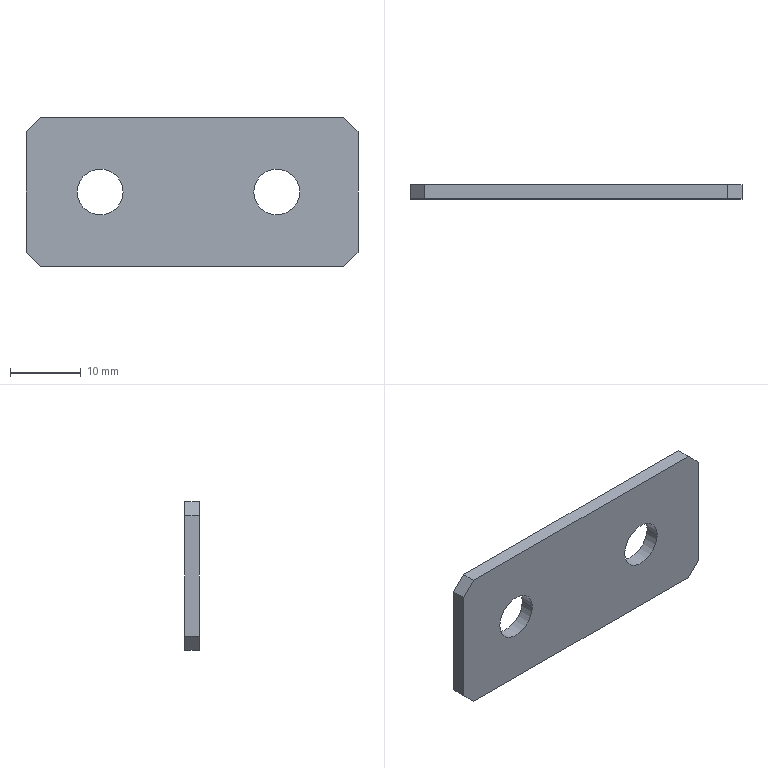Component | SolidWorks | Crossbeam.1(Item52)-1_Block-1 | 1 solid | 14 faces | box 47 x 2 x 21 mm | volume 1825 mm3 | plane 10 | cylinder 4 | commonest cylinder face diameters 6.5 x4 | material Plain Carbon Steel
STEP:
#1=COLOUR_RGB('',0.7922,0.8196,0.9333);
#2=FILL_AREA_STYLE_COLOUR('',#1);
#3=FILL_AREA_STYLE('',(#2));
#4=SURFACE_STYLE_FILL_AREA(#3);
#5=SURFACE_SIDE_STYLE('',(#4));
#6=SURFACE_STYLE_USAGE(.BOTH.,#5);
#7=PRESENTATION_STYLE_ASSIGNMENT((#6));
#8=CARTESIAN_POINT('',(-15.384,14.764,-43.799));
#9=VERTEX_POINT('',#8);
#10=CARTESIAN_POINT('',(-15.128,14.764,-43.799));
#11=VERTEX_POINT('',#10);
#12=CARTESIAN_POINT('',(-15.256,14.764,-43.799));
#13=DIRECTION('',(0.,-1.,-0.));
#14=DIRECTION('',(1.,0.,0.));
#15=AXIS2_PLACEMENT_3D('',#12,#13,#14);
#16=CIRCLE('',#15,0.128);
#17=EDGE_CURVE('',#9,#11,#16,.T.);
#18=ORIENTED_EDGE('',*,*,#17,.F.);
#19=CARTESIAN_POINT('',(-15.384,14.685,-43.799));
#20=VERTEX_POINT('',#19);
#21=CARTESIAN_POINT('',(-15.384,14.764,-43.799));
#22=DIRECTION('',(0.,-1.,-0.));
#23=VECTOR('',#22,39.37);
#24=LINE('',#21,#23);
#25=EDGE_CURVE('',#9,#20,#24,.T.);
#26=ORIENTED_EDGE('',*,*,#25,.T.);
#27=CARTESIAN_POINT('',(-15.128,14.685,-43.799));
#28=VERTEX_POINT('',#27);
#29=CARTESIAN_POINT('',(-15.256,14.685,-43.799));
#30=DIRECTION('',(0.,-1.,-0.));
#31=DIRECTION('',(1.,0.,0.));
#32=AXIS2_PLACEMENT_3D('',#29,#30,#31);
#33=CIRCLE('',#32,0.128);
#34=EDGE_CURVE('',#20,#28,#33,.T.);
#35=ORIENTED_EDGE('',*,*,#34,.T.);
#36=CARTESIAN_POINT('',(-15.128,14.764,-43.799));
#37=DIRECTION('',(0.,-1.,-0.));
#38=VECTOR('',#37,39.37);
#39=LINE('',#36,#38);
#40=EDGE_CURVE('',#11,#28,#39,.T.);
#41=ORIENTED_EDGE('',*,*,#40,.F.);
#42=EDGE_LOOP('',(#18,#26,#35,#41));
#43=FACE_OUTER_BOUND('',#42,.T.);
#44=CARTESIAN_POINT('',(-15.256,14.764,-43.799));
#45=DIRECTION('',(0.,-1.,-0.));
#46=DIRECTION('',(1.,0.,0.));
#47=AXIS2_PLACEMENT_3D('',#44,#45,#46);
#48=CYLINDRICAL_SURFACE('',#47,0.128);
#49=ADVANCED_FACE('',(#43),#48,.F.);
#50=CARTESIAN_POINT('',(-14.4,14.764,-43.799));
#51=VERTEX_POINT('',#50);
#52=CARTESIAN_POINT('',(-14.144,14.764,-43.799));
#53=VERTEX_POINT('',#52);
#54=CARTESIAN_POINT('',(-14.272,14.764,-43.799));
#55=DIRECTION('',(0.,-1.,-0.));
#56=DIRECTION('',(1.,0.,0.));
#57=AXIS2_PLACEMENT_3D('',#54,#55,#56);
#58=CIRCLE('',#57,0.128);
#59=EDGE_CURVE('',#51,#53,#58,.T.);
#60=ORIENTED_EDGE('',*,*,#59,.F.);
#61=CARTESIAN_POINT('',(-14.4,14.685,-43.799));
#62=VERTEX_POINT('',#61);
#63=CARTESIAN_POINT('',(-14.4,14.764,-43.799));
#64=DIRECTION('',(0.,-1.,-0.));
#65=VECTOR('',#64,39.37);
#66=LINE('',#63,#65);
#67=EDGE_CURVE('',#51,#62,#66,.T.);
#68=ORIENTED_EDGE('',*,*,#67,.T.);
#69=CARTESIAN_POINT('',(-14.144,14.685,-43.799));
#70=VERTEX_POINT('',#69);
#71=CARTESIAN_POINT('',(-14.272,14.685,-43.799));
#72=DIRECTION('',(0.,-1.,-0.));
#73=DIRECTION('',(1.,0.,0.));
#74=AXIS2_PLACEMENT_3D('',#71,#72,#73);
#75=CIRCLE('',#74,0.128);
#76=EDGE_CURVE('',#62,#70,#75,.T.);
#77=ORIENTED_EDGE('',*,*,#76,.T.);
#78=CARTESIAN_POINT('',(-14.144,14.764,-43.799));
#79=DIRECTION('',(0.,-1.,-0.));
#80=VECTOR('',#79,39.37);
#81=LINE('',#78,#80);
#82=EDGE_CURVE('',#53,#70,#81,.T.);
#83=ORIENTED_EDGE('',*,*,#82,.F.);
#84=EDGE_LOOP('',(#60,#68,#77,#83));
#85=FACE_OUTER_BOUND('',#84,.T.);
#86=CARTESIAN_POINT('',(-14.272,14.764,-43.799));
#87=DIRECTION('',(0.,-1.,-0.));
#88=DIRECTION('',(1.,0.,0.));
#89=AXIS2_PLACEMENT_3D('',#86,#87,#88);
#90=CYLINDRICAL_SURFACE('',#89,0.128);
#91=ADVANCED_FACE('',(#85),#90,.F.);
#92=CARTESIAN_POINT('',(-13.819,14.764,-44.134));
#93=VERTEX_POINT('',#92);
#94=CARTESIAN_POINT('',(-13.819,14.764,-43.465));
#95=VERTEX_POINT('',#94);
#96=CARTESIAN_POINT('',(-13.819,14.764,-44.213));
#97=DIRECTION('',(-0.,-0.,1.));
#98=VECTOR('',#97,39.37);
#99=LINE('',#96,#98);
#100=EDGE_CURVE('',#93,#95,#99,.T.);
#101=ORIENTED_EDGE('',*,*,#100,.T.);
#102=CARTESIAN_POINT('',(-13.819,14.685,-43.465));
#103=VERTEX_POINT('',#102);
#104=CARTESIAN_POINT('',(-13.819,14.764,-43.465));
#105=DIRECTION('',(0.,-1.,-0.));
#106=VECTOR('',#105,39.37);
#107=LINE('',#104,#106);
#108=EDGE_CURVE('',#95,#103,#107,.T.);
#109=ORIENTED_EDGE('',*,*,#108,.T.);
#110=CARTESIAN_POINT('',(-13.819,14.685,-44.134));
#111=VERTEX_POINT('',#110);
#112=CARTESIAN_POINT('',(-13.819,14.685,-44.213));
#113=DIRECTION('',(-0.,-0.,1.));
#114=VECTOR('',#113,39.37);
#115=LINE('',#112,#114);
#116=EDGE_CURVE('',#111,#103,#115,.T.);
#117=ORIENTED_EDGE('',*,*,#116,.F.);
#118=CARTESIAN_POINT('',(-13.819,14.764,-44.134));
#119=DIRECTION('',(-0.,1.,0.));
#120=VECTOR('',#119,39.37);
#121=LINE('',#118,#120);
#122=EDGE_CURVE('',#111,#93,#121,.T.);
#123=ORIENTED_EDGE('',*,*,#122,.T.);
#124=EDGE_LOOP('',(#101,#109,#117,#123));
#125=FACE_OUTER_BOUND('',#124,.T.);
#126=CARTESIAN_POINT('',(-13.819,14.764,-44.213));
#127=DIRECTION('',(1.,0.,0.));
#128=DIRECTION('',(-0.,1.,0.));
#129=AXIS2_PLACEMENT_3D('',#126,#127,#128);
#130=PLANE('',#129);
#131=ADVANCED_FACE('',(#125),#130,.T.);
#132=CARTESIAN_POINT('',(-15.591,14.685,-44.213));
#133=VERTEX_POINT('',#132);
#134=CARTESIAN_POINT('',(-13.898,14.685,-44.213));
#135=VERTEX_POINT('',#134);
#136=CARTESIAN_POINT('',(-15.669,14.685,-44.213));
#137=DIRECTION('',(1.,0.,0.));
#138=VECTOR('',#137,39.37);
#139=LINE('',#136,#138);
#140=EDGE_CURVE('',#133,#135,#139,.T.);
#141=ORIENTED_EDGE('',*,*,#140,.F.);
#142=CARTESIAN_POINT('',(-15.591,14.764,-44.213));
#143=VERTEX_POINT('',#142);
#144=CARTESIAN_POINT('',(-15.591,14.764,-44.213));
#145=DIRECTION('',(-0.,1.,0.));
#146=VECTOR('',#145,39.37);
#147=LINE('',#144,#146);
#148=EDGE_CURVE('',#133,#143,#147,.T.);
#149=ORIENTED_EDGE('',*,*,#148,.T.);
#150=CARTESIAN_POINT('',(-13.898,14.764,-44.213));
#151=VERTEX_POINT('',#150);
#152=CARTESIAN_POINT('',(-15.669,14.764,-44.213));
#153=DIRECTION('',(1.,0.,0.));
#154=VECTOR('',#153,39.37);
#155=LINE('',#152,#154);
#156=EDGE_CURVE('',#143,#151,#155,.T.);
#157=ORIENTED_EDGE('',*,*,#156,.T.);
#158=CARTESIAN_POINT('',(-13.898,14.764,-44.213));
#159=DIRECTION('',(0.,-1.,-0.));
#160=VECTOR('',#159,39.37);
#161=LINE('',#158,#160);
#162=EDGE_CURVE('',#151,#135,#161,.T.);
#163=ORIENTED_EDGE('',*,*,#162,.T.);
#164=EDGE_LOOP('',(#141,#149,#157,#163));
#165=FACE_OUTER_BOUND('',#164,.T.);
#166=CARTESIAN_POINT('',(-15.669,14.764,-44.213));
#167=DIRECTION('',(0.,0.,-1.));
#168=DIRECTION('',(-0.,1.,0.));
#169=AXIS2_PLACEMENT_3D('',#166,#167,#168);
#170=PLANE('',#169);
#171=ADVANCED_FACE('',(#165),#170,.T.);
#172=CARTESIAN_POINT('',(-15.669,14.685,-43.465));
#173=VERTEX_POINT('',#172);
#174=CARTESIAN_POINT('',(-15.669,14.685,-44.134));
#175=VERTEX_POINT('',#174);
#176=CARTESIAN_POINT('',(-15.669,14.685,-44.213));
#177=DIRECTION('',(0.,0.,-1.));
#178=VECTOR('',#177,39.37);
#179=LINE('',#176,#178);
#180=EDGE_CURVE('',#173,#175,#179,.T.);
#181=ORIENTED_EDGE('',*,*,#180,.F.);
#182=CARTESIAN_POINT('',(-15.669,14.764,-43.465));
#183=VERTEX_POINT('',#182);
#184=CARTESIAN_POINT('',(-15.669,14.764,-43.465));
#185=DIRECTION('',(-0.,1.,0.));
#186=VECTOR('',#185,39.37);
#187=LINE('',#184,#186);
#188=EDGE_CURVE('',#173,#183,#187,.T.);
#189=ORIENTED_EDGE('',*,*,#188,.T.);
#190=CARTESIAN_POINT('',(-15.669,14.764,-44.134));
#191=VERTEX_POINT('',#190);
#192=CARTESIAN_POINT('',(-15.669,14.764,-44.213));
#193=DIRECTION('',(0.,0.,-1.));
#194=VECTOR('',#193,39.37);
#195=LINE('',#192,#194);
#196=EDGE_CURVE('',#183,#191,#195,.T.);
#197=ORIENTED_EDGE('',*,*,#196,.T.);
#198=CARTESIAN_POINT('',(-15.669,14.764,-44.134));
#199=DIRECTION('',(0.,-1.,-0.));
#200=VECTOR('',#199,39.37);
#201=LINE('',#198,#200);
#202=EDGE_CURVE('',#191,#175,#201,.T.);
#203=ORIENTED_EDGE('',*,*,#202,.T.);
#204=EDGE_LOOP('',(#181,#189,#197,#203));
#205=FACE_OUTER_BOUND('',#204,.T.);
#206=CARTESIAN_POINT('',(-15.669,14.764,-44.213));
#207=DIRECTION('',(-1.,-0.,-0.));
#208=DIRECTION('',(0.,-1.,-0.));
#209=AXIS2_PLACEMENT_3D('',#206,#207,#208);
#210=PLANE('',#209);
#211=ADVANCED_FACE('',(#205),#210,.T.);
#212=CARTESIAN_POINT('',(-13.898,14.764,-43.386));
#213=VERTEX_POINT('',#212);
#214=CARTESIAN_POINT('',(-15.591,14.764,-43.386));
#215=VERTEX_POINT('',#214);
#216=CARTESIAN_POINT('',(-15.669,14.764,-43.386));
#217=DIRECTION('',(-1.,-0.,-0.));
#218=VECTOR('',#217,39.37);
#219=LINE('',#216,#218);
#220=EDGE_CURVE('',#213,#215,#219,.T.);
#221=ORIENTED_EDGE('',*,*,#220,.T.);
#222=CARTESIAN_POINT('',(-15.591,14.685,-43.386));
#223=VERTEX_POINT('',#222);
#224=CARTESIAN_POINT('',(-15.591,14.764,-43.386));
#225=DIRECTION('',(0.,-1.,-0.));
#226=VECTOR('',#225,39.37);
#227=LINE('',#224,#226);
#228=EDGE_CURVE('',#215,#223,#227,.T.);
#229=ORIENTED_EDGE('',*,*,#228,.T.);
#230=CARTESIAN_POINT('',(-13.898,14.685,-43.386));
#231=VERTEX_POINT('',#230);
#232=CARTESIAN_POINT('',(-15.669,14.685,-43.386));
#233=DIRECTION('',(-1.,-0.,-0.));
#234=VECTOR('',#233,39.37);
#235=LINE('',#232,#234);
#236=EDGE_CURVE('',#231,#223,#235,.T.);
#237=ORIENTED_EDGE('',*,*,#236,.F.);
#238=CARTESIAN_POINT('',(-13.898,14.764,-43.386));
#239=DIRECTION('',(-0.,1.,0.));
#240=VECTOR('',#239,39.37);
#241=LINE('',#238,#240);
#242=EDGE_CURVE('',#231,#213,#241,.T.);
#243=ORIENTED_EDGE('',*,*,#242,.T.);
#244=EDGE_LOOP('',(#221,#229,#237,#243));
#245=FACE_OUTER_BOUND('',#244,.T.);
#246=CARTESIAN_POINT('',(-15.669,14.764,-43.386));
#247=DIRECTION('',(-0.,-0.,1.));
#248=DIRECTION('',(0.,-1.,-0.));
#249=AXIS2_PLACEMENT_3D('',#246,#247,#248);
#250=PLANE('',#249);
#251=ADVANCED_FACE('',(#245),#250,.T.);
#252=CARTESIAN_POINT('',(-15.256,14.764,-43.799));
#253=DIRECTION('',(0.,-1.,-0.));
#254=DIRECTION('',(1.,0.,0.));
#255=AXIS2_PLACEMENT_3D('',#252,#253,#254);
#256=CIRCLE('',#255,0.128);
#257=EDGE_CURVE('',#11,#9,#256,.T.);
#258=ORIENTED_EDGE('',*,*,#257,.T.);
#259=ORIENTED_EDGE('',*,*,#17,.T.);
#260=EDGE_LOOP('',(#258,#259));
#261=FACE_BOUND('',#260,.T.);
#262=CARTESIAN_POINT('',(-14.272,14.764,-43.799));
#263=DIRECTION('',(0.,-1.,-0.));
#264=DIRECTION('',(1.,0.,0.));
#265=AXIS2_PLACEMENT_3D('',#262,#263,#264);
#266=CIRCLE('',#265,0.128);
#267=EDGE_CURVE('',#53,#51,#266,.T.);
#268=ORIENTED_EDGE('',*,*,#267,.T.);
#269=ORIENTED_EDGE('',*,*,#59,.T.);
#270=EDGE_LOOP('',(#268,#269));
#271=FACE_BOUND('',#270,.T.);
#272=ORIENTED_EDGE('',*,*,#196,.F.);
#273=CARTESIAN_POINT('',(-14.705,14.764,-42.5));
#274=DIRECTION('',(0.7071,0.,0.7071));
#275=VECTOR('',#274,39.37);
#276=LINE('',#273,#275);
#277=EDGE_CURVE('',#183,#215,#276,.T.);
#278=ORIENTED_EDGE('',*,*,#277,.T.);
#279=ORIENTED_EDGE('',*,*,#220,.F.);
#280=CARTESIAN_POINT('',(-13.858,14.764,-43.425));
#281=DIRECTION('',(0.7071,0.,-0.7071));
#282=VECTOR('',#281,39.37);
#283=LINE('',#280,#282);
#284=EDGE_CURVE('',#213,#95,#283,.T.);
#285=ORIENTED_EDGE('',*,*,#284,.T.);
#286=ORIENTED_EDGE('',*,*,#100,.F.);
#287=CARTESIAN_POINT('',(-13.445,14.764,-43.76));
#288=DIRECTION('',(-0.7071,-0.,-0.7071));
#289=VECTOR('',#288,39.37);
#290=LINE('',#287,#289);
#291=EDGE_CURVE('',#93,#151,#290,.T.);
#292=ORIENTED_EDGE('',*,*,#291,.T.);
#293=ORIENTED_EDGE('',*,*,#156,.F.);
#294=CARTESIAN_POINT('',(-15.118,14.764,-44.685));
#295=DIRECTION('',(-0.7071,-0.,0.7071));
#296=VECTOR('',#295,39.37);
#297=LINE('',#294,#296);
#298=EDGE_CURVE('',#143,#191,#297,.T.);
#299=ORIENTED_EDGE('',*,*,#298,.T.);
#300=EDGE_LOOP('',(#272,#278,#279,#285,#286,#292,#293,#299));
#301=FACE_OUTER_BOUND('',#300,.T.);
#302=CARTESIAN_POINT('',(-13.819,14.764,-43.386));
#303=DIRECTION('',(-0.,1.,0.));
#304=DIRECTION('',(-1.,-0.,-0.));
#305=AXIS2_PLACEMENT_3D('',#302,#303,#304);
#306=PLANE('',#305);
#307=ADVANCED_FACE('',(#261,#271,#301),#306,.T.);
#308=CARTESIAN_POINT('',(-15.256,14.685,-43.799));
#309=DIRECTION('',(0.,-1.,-0.));
#310=DIRECTION('',(1.,0.,0.));
#311=AXIS2_PLACEMENT_3D('',#308,#309,#310);
#312=CIRCLE('',#311,0.128);
#313=EDGE_CURVE('',#28,#20,#312,.T.);
#314=ORIENTED_EDGE('',*,*,#313,.F.);
#315=ORIENTED_EDGE('',*,*,#34,.F.);
#316=EDGE_LOOP('',(#314,#315));
#317=FACE_BOUND('',#316,.T.);
#318=CARTESIAN_POINT('',(-14.272,14.685,-43.799));
#319=DIRECTION('',(0.,-1.,-0.));
#320=DIRECTION('',(1.,0.,0.));
#321=AXIS2_PLACEMENT_3D('',#318,#319,#320);
#322=CIRCLE('',#321,0.128);
#323=EDGE_CURVE('',#70,#62,#322,.T.);
#324=ORIENTED_EDGE('',*,*,#323,.F.);
#325=ORIENTED_EDGE('',*,*,#76,.F.);
#326=EDGE_LOOP('',(#324,#325));
#327=FACE_BOUND('',#326,.T.);
#328=ORIENTED_EDGE('',*,*,#236,.T.);
#329=CARTESIAN_POINT('',(-15.591,14.685,-43.386));
#330=DIRECTION('',(-0.7071,-0.,-0.7071));
#331=VECTOR('',#330,39.37);
#332=LINE('',#329,#331);
#333=EDGE_CURVE('',#223,#173,#332,.T.);
#334=ORIENTED_EDGE('',*,*,#333,.T.);
#335=ORIENTED_EDGE('',*,*,#180,.T.);
#336=CARTESIAN_POINT('',(-15.669,14.685,-44.134));
#337=DIRECTION('',(0.7071,0.,-0.7071));
#338=VECTOR('',#337,39.37);
#339=LINE('',#336,#338);
#340=EDGE_CURVE('',#175,#133,#339,.T.);
#341=ORIENTED_EDGE('',*,*,#340,.T.);
#342=ORIENTED_EDGE('',*,*,#140,.T.);
#343=CARTESIAN_POINT('',(-13.898,14.685,-44.213));
#344=DIRECTION('',(0.7071,0.,0.7071));
#345=VECTOR('',#344,39.37);
#346=LINE('',#343,#345);
#347=EDGE_CURVE('',#135,#111,#346,.T.);
#348=ORIENTED_EDGE('',*,*,#347,.T.);
#349=ORIENTED_EDGE('',*,*,#116,.T.);
#350=CARTESIAN_POINT('',(-13.819,14.685,-43.465));
#351=DIRECTION('',(-0.7071,-0.,0.7071));
#352=VECTOR('',#351,39.37);
#353=LINE('',#350,#352);
#354=EDGE_CURVE('',#103,#231,#353,.T.);
#355=ORIENTED_EDGE('',*,*,#354,.T.);
#356=EDGE_LOOP('',(#328,#334,#335,#341,#342,#348,#349,#355));
#357=FACE_OUTER_BOUND('',#356,.T.);
#358=CARTESIAN_POINT('',(-13.819,14.685,-43.386));
#359=DIRECTION('',(-0.,1.,0.));
#360=DIRECTION('',(-1.,-0.,-0.));
#361=AXIS2_PLACEMENT_3D('',#358,#359,#360);
#362=PLANE('',#361);
#363=ADVANCED_FACE('',(#317,#327,#357),#362,.F.);
#364=ORIENTED_EDGE('',*,*,#67,.F.);
#365=ORIENTED_EDGE('',*,*,#267,.F.);
#366=ORIENTED_EDGE('',*,*,#82,.T.);
#367=ORIENTED_EDGE('',*,*,#323,.T.);
#368=EDGE_LOOP('',(#364,#365,#366,#367));
#369=FACE_OUTER_BOUND('',#368,.T.);
#370=CARTESIAN_POINT('',(-14.272,14.764,-43.799));
#371=DIRECTION('',(0.,-1.,-0.));
#372=DIRECTION('',(1.,0.,0.));
#373=AXIS2_PLACEMENT_3D('',#370,#371,#372);
#374=CYLINDRICAL_SURFACE('',#373,0.128);
#375=ADVANCED_FACE('',(#369),#374,.F.);
#376=ORIENTED_EDGE('',*,*,#25,.F.);
#377=ORIENTED_EDGE('',*,*,#257,.F.);
#378=ORIENTED_EDGE('',*,*,#40,.T.);
#379=ORIENTED_EDGE('',*,*,#313,.T.);
#380=EDGE_LOOP('',(#376,#377,#378,#379));
#381=FACE_OUTER_BOUND('',#380,.T.);
#382=CARTESIAN_POINT('',(-15.256,14.764,-43.799));
#383=DIRECTION('',(0.,-1.,-0.));
#384=DIRECTION('',(1.,0.,0.));
#385=AXIS2_PLACEMENT_3D('',#382,#383,#384);
#386=CYLINDRICAL_SURFACE('',#385,0.128);
#387=ADVANCED_FACE('',(#381),#386,.F.);
#388=ORIENTED_EDGE('',*,*,#277,.F.);
#389=ORIENTED_EDGE('',*,*,#188,.F.);
#390=ORIENTED_EDGE('',*,*,#333,.F.);
#391=ORIENTED_EDGE('',*,*,#228,.F.);
#392=EDGE_LOOP('',(#388,#389,#390,#391));
#393=FACE_OUTER_BOUND('',#392,.T.);
#394=CARTESIAN_POINT('',(-15.591,14.764,-43.386));
#395=DIRECTION('',(0.7071,0.,-0.7071));
#396=DIRECTION('',(0.7071,0.,0.7071));
#397=AXIS2_PLACEMENT_3D('',#394,#395,#396);
#398=PLANE('',#397);
#399=ADVANCED_FACE('',(#393),#398,.F.);
#400=ORIENTED_EDGE('',*,*,#298,.F.);
#401=ORIENTED_EDGE('',*,*,#148,.F.);
#402=ORIENTED_EDGE('',*,*,#340,.F.);
#403=ORIENTED_EDGE('',*,*,#202,.F.);
#404=EDGE_LOOP('',(#400,#401,#402,#403));
#405=FACE_OUTER_BOUND('',#404,.T.);
#406=CARTESIAN_POINT('',(-15.669,14.764,-44.134));
#407=DIRECTION('',(0.7071,0.,0.7071));
#408=DIRECTION('',(-0.7071,-0.,0.7071));
#409=AXIS2_PLACEMENT_3D('',#406,#407,#408);
#410=PLANE('',#409);
#411=ADVANCED_FACE('',(#405),#410,.F.);
#412=ORIENTED_EDGE('',*,*,#284,.F.);
#413=ORIENTED_EDGE('',*,*,#242,.F.);
#414=ORIENTED_EDGE('',*,*,#354,.F.);
#415=ORIENTED_EDGE('',*,*,#108,.F.);
#416=EDGE_LOOP('',(#412,#413,#414,#415));
#417=FACE_OUTER_BOUND('',#416,.T.);
#418=CARTESIAN_POINT('',(-13.819,14.764,-43.465));
#419=DIRECTION('',(-0.7071,-0.,-0.7071));
#420=DIRECTION('',(0.7071,0.,-0.7071));
#421=AXIS2_PLACEMENT_3D('',#418,#419,#420);
#422=PLANE('',#421);
#423=ADVANCED_FACE('',(#417),#422,.F.);
#424=ORIENTED_EDGE('',*,*,#291,.F.);
#425=ORIENTED_EDGE('',*,*,#122,.F.);
#426=ORIENTED_EDGE('',*,*,#347,.F.);
#427=ORIENTED_EDGE('',*,*,#162,.F.);
#428=EDGE_LOOP('',(#424,#425,#426,#427));
#429=FACE_OUTER_BOUND('',#428,.T.);
#430=CARTESIAN_POINT('',(-13.898,14.764,-44.213));
#431=DIRECTION('',(-0.7071,-0.,0.7071));
#432=DIRECTION('',(-0.7071,-0.,-0.7071));
#433=AXIS2_PLACEMENT_3D('',#430,#431,#432);
#434=PLANE('',#433);
#435=ADVANCED_FACE('',(#429),#434,.F.);
#436=CLOSED_SHELL('',(#49,#91,#131,#171,#211,#251,#307,#363,#375,#387,#399,#411,#423,#435));
#437=MANIFOLD_SOLID_BREP('',#436);
#438=STYLED_ITEM('',(#7),#437);
#439=PRESENTATION_LAYER_ASSIGNMENT('','',(#438));
#440=CARTESIAN_POINT('',(0.,0.,0.));
#441=DIRECTION('',(0.,0.,1.));
#442=DIRECTION('',(1.,0.,0.));
#443=AXIS2_PLACEMENT_3D('',#440,#441,#442);
#444=(LENGTH_UNIT()NAMED_UNIT(*)SI_UNIT($,.METRE.));
#445=LENGTH_MEASURE_WITH_UNIT(LENGTH_MEASURE(0.0254),#444);
#446=DIMENSIONAL_EXPONENTS(1.,0.,0.,0.,0.,0.,0.);
#447=(CONVERSION_BASED_UNIT('',#445)LENGTH_UNIT()NAMED_UNIT(#446));
#448=UNCERTAINTY_MEASURE_WITH_UNIT(LENGTH_MEASURE(0.00001),#447,'','');
#449=(NAMED_UNIT(*)PLANE_ANGLE_UNIT()SI_UNIT($,.RADIAN.));
#450=(NAMED_UNIT(*)SI_UNIT($,.STERADIAN.)SOLID_ANGLE_UNIT());
#451=(GEOMETRIC_REPRESENTATION_CONTEXT(3)GLOBAL_UNCERTAINTY_ASSIGNED_CONTEXT((#448))GLOBAL_UNIT_ASSIGNED_CONTEXT((#447,#449,#450))REPRESENTATION_CONTEXT('',''));
#452=ADVANCED_BREP_SHAPE_REPRESENTATION('',(#437,#443),#451);
#453=(LENGTH_UNIT()NAMED_UNIT(*)SI_UNIT($,.METRE.));
#454=LENGTH_MEASURE_WITH_UNIT(LENGTH_MEASURE(0.0254),#453);
#455=DIMENSIONAL_EXPONENTS(1.,0.,0.,0.,0.,0.,0.);
#456=(CONVERSION_BASED_UNIT('',#454)LENGTH_UNIT()NAMED_UNIT(#455));
#457=UNCERTAINTY_MEASURE_WITH_UNIT(LENGTH_MEASURE(0.00001),#456,'','');
#458=(NAMED_UNIT(*)PLANE_ANGLE_UNIT()SI_UNIT($,.RADIAN.));
#459=(NAMED_UNIT(*)SI_UNIT($,.STERADIAN.)SOLID_ANGLE_UNIT());
#460=(GEOMETRIC_REPRESENTATION_CONTEXT(3)GLOBAL_UNCERTAINTY_ASSIGNED_CONTEXT((#457))GLOBAL_UNIT_ASSIGNED_CONTEXT((#456,#458,#459))REPRESENTATION_CONTEXT('',''));
#461=MECHANICAL_DESIGN_GEOMETRIC_PRESENTATION_REPRESENTATION('',(#438),#460);